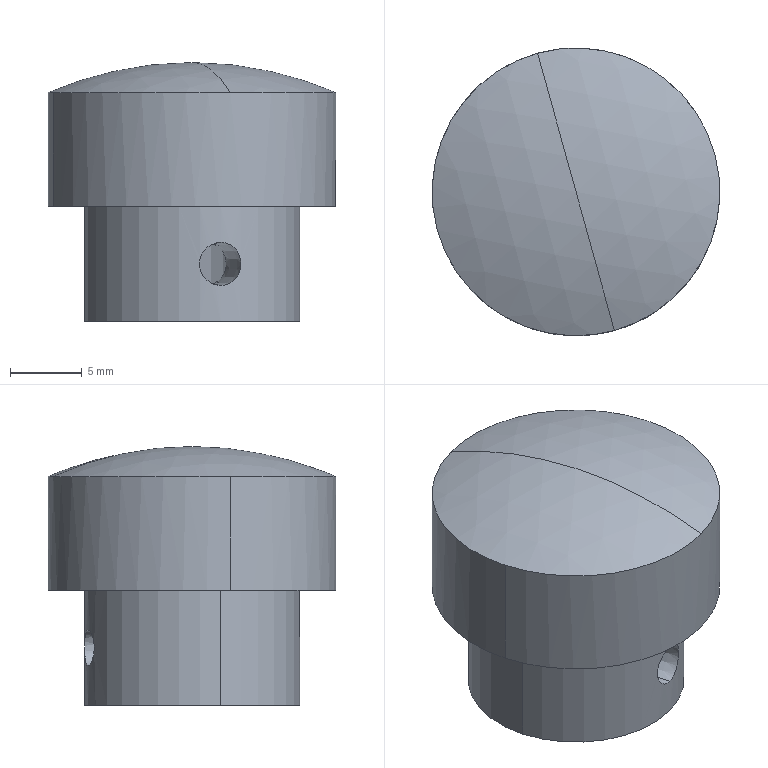Component | SolidWorks | 17Handle-1 | 1 solid | 16 faces | box 20 x 20 x 18 mm | volume 3748 mm3 | cone 6 | cylinder 6 | sphere 2 | plane 2 | commonest cylinder face diameters 8 x2 15 x2 20 x2
build123d program:
from build123d import *

# Parameters (mm, degrees)
SIZE_MM_DOWEL_PIN_HOLE1_D     = 8
SIZE_MM_DOWEL_PIN_HOLE1_DEPTH = 8
SIZE_MM_DOWEL_PIN_HOLE1_TIP   = 2.403


with BuildPart() as part:
    # Sketch6 → Revolve1 (revolve)
    with BuildSketch(Plane(origin=(0, 0, 0), x_dir=(0, 0, -1), z_dir=(1, 0, 0)), mode=Mode.PRIVATE) as revolve1_sk:
        with BuildLine():
            Line((-2.087, 10), (-10, 10))
            Line((-10, 10), (-10, 7.5))
            Line((-10, 7.5), (-18, 7.5))
            Line((-18, 7.5), (-18, 0))
            Line((-18, 0), (0, 0))
            ThreePointArc((0, 0), (-0.5273, 5.108), (-2.087, 10))
        make_face()
    revolve(revolve1_sk.sketch.rotate(Axis((0, 0, 0), (0, 0, 1)), 90), axis=Axis((0, 0, 0), (0, 0, 1)))

    # Size mm Dowel Pin Hole1
    with Locations(Plane.XY.offset(18)):
        with Locations((0, 0)):
            Hole(SIZE_MM_DOWEL_PIN_HOLE1_D / 2, depth=SIZE_MM_DOWEL_PIN_HOLE1_DEPTH)
            with Locations((0, 0, -(SIZE_MM_DOWEL_PIN_HOLE1_DEPTH + SIZE_MM_DOWEL_PIN_HOLE1_TIP / 2))):  # 118° drill point
                Cone(0, SIZE_MM_DOWEL_PIN_HOLE1_D / 2, SIZE_MM_DOWEL_PIN_HOLE1_TIP, mode=Mode.SUBTRACT)

    # Cut-Extrude2 cone 1 section (on through the dimple's axis) → Cut-Extrude2 (revolve, cut)
    with BuildSketch(Plane(origin=(0, 7.5, 14), x_dir=(0, 0, 1), z_dir=(1, 0, 0))):
        Polygon((0, 0), (1.5, 0), (0, 85.935), align=None)
    revolve(axis=Axis((0, 7.5, 14), (0, -1, 0)), mode=Mode.SUBTRACT)


solid = part.part

# Placed as in the assembly
solid = solid.moved(Location((33.957, 1.776, 451), (180, 0, -15.474)))
STEP:
#1=COLOUR_RGB('',0.7922,0.8196,0.9333);
#2=FILL_AREA_STYLE_COLOUR('',#1);
#3=FILL_AREA_STYLE('',(#2));
#4=SURFACE_STYLE_FILL_AREA(#3);
#5=SURFACE_SIDE_STYLE('',(#4));
#6=SURFACE_STYLE_USAGE(.BOTH.,#5);
#7=PRESENTATION_STYLE_ASSIGNMENT((#6));
#8=CARTESIAN_POINT('',(1.258,0.3545,17.156));
#9=VERTEX_POINT('',#8);
#10=CARTESIAN_POINT('',(1.258,0.3545,17.253));
#11=VERTEX_POINT('',#10);
#12=CARTESIAN_POINT('',(1.258,0.3545,17.156));
#13=CARTESIAN_POINT('',(1.252,0.3528,17.156));
#14=CARTESIAN_POINT('',(1.246,0.3509,17.157));
#15=CARTESIAN_POINT('',(1.235,0.347,17.162));
#16=CARTESIAN_POINT('',(1.23,0.3451,17.166));
#17=CARTESIAN_POINT('',(1.223,0.3425,17.173));
#18=CARTESIAN_POINT('',(1.221,0.3417,17.175));
#19=CARTESIAN_POINT('',(1.218,0.3403,17.18));
#20=CARTESIAN_POINT('',(1.217,0.3396,17.183));
#21=CARTESIAN_POINT('',(1.213,0.3381,17.192));
#22=CARTESIAN_POINT('',(1.212,0.3376,17.198));
#23=CARTESIAN_POINT('',(1.212,0.3375,17.211));
#24=CARTESIAN_POINT('',(1.213,0.3381,17.217));
#25=CARTESIAN_POINT('',(1.218,0.3401,17.229));
#26=CARTESIAN_POINT('',(1.221,0.3416,17.235));
#27=CARTESIAN_POINT('',(1.228,0.3442,17.241));
#28=CARTESIAN_POINT('',(1.23,0.3451,17.243));
#29=CARTESIAN_POINT('',(1.235,0.347,17.247));
#30=CARTESIAN_POINT('',(1.237,0.348,17.249));
#31=CARTESIAN_POINT('',(1.246,0.3509,17.252));
#32=CARTESIAN_POINT('',(1.252,0.3528,17.253));
#33=CARTESIAN_POINT('',(1.258,0.3545,17.253));
#34=B_SPLINE_CURVE_WITH_KNOTS('',3,(#12,#13,#14,#15,#16,#17,#18,#19,#20,#21,#22,#23,#24,#25,#26,#27,#28,#29,#30,#31,#32,#33),.UNSPECIFIED.,.F.,.F.,(4,2,2,2,2,2,2,2,2,2,4),(0.004899,0.005384,0.005868,0.006111,0.006353,0.006838,0.007323,0.007808,0.00805,0.008293,0.008778),.UNSPECIFIED.);
#35=EDGE_CURVE('',#9,#11,#34,.T.);
#36=ORIENTED_EDGE('',*,*,#35,.T.);
#37=CARTESIAN_POINT('',(1.295,0.2217,17.256));
#38=VERTEX_POINT('',#37);
#39=CARTESIAN_POINT('',(1.416,-0.2146,17.264));
#40=DIRECTION('',(0.2668,-0.9636,0.01745));
#41=VECTOR('',#40,39.37);
#42=LINE('',#39,#41);
#43=EDGE_CURVE('',#11,#38,#42,.T.);
#44=ORIENTED_EDGE('',*,*,#43,.T.);
#45=CARTESIAN_POINT('',(1.295,0.2217,17.154));
#46=VERTEX_POINT('',#45);
#47=CARTESIAN_POINT('',(1.295,0.2217,17.154));
#48=CARTESIAN_POINT('',(1.292,0.2208,17.154));
#49=CARTESIAN_POINT('',(1.288,0.2198,17.154));
#50=CARTESIAN_POINT('',(1.282,0.2176,17.155));
#51=CARTESIAN_POINT('',(1.279,0.2164,17.156));
#52=CARTESIAN_POINT('',(1.27,0.2128,17.16));
#53=CARTESIAN_POINT('',(1.265,0.2103,17.164));
#54=CARTESIAN_POINT('',(1.257,0.2056,17.173));
#55=CARTESIAN_POINT('',(1.253,0.2035,17.179));
#56=CARTESIAN_POINT('',(1.249,0.2006,17.191));
#57=CARTESIAN_POINT('',(1.248,0.1997,17.198));
#58=CARTESIAN_POINT('',(1.248,0.1997,17.208));
#59=CARTESIAN_POINT('',(1.248,0.1999,17.211));
#60=CARTESIAN_POINT('',(1.249,0.2007,17.218));
#61=CARTESIAN_POINT('',(1.25,0.2013,17.221));
#62=CARTESIAN_POINT('',(1.253,0.2035,17.231));
#63=CARTESIAN_POINT('',(1.257,0.2056,17.236));
#64=CARTESIAN_POINT('',(1.263,0.2091,17.243));
#65=CARTESIAN_POINT('',(1.266,0.2103,17.245));
#66=CARTESIAN_POINT('',(1.271,0.2128,17.249));
#67=CARTESIAN_POINT('',(1.273,0.2141,17.251));
#68=CARTESIAN_POINT('',(1.282,0.2177,17.255));
#69=CARTESIAN_POINT('',(1.288,0.2199,17.256));
#70=CARTESIAN_POINT('',(1.295,0.2217,17.256));
#71=B_SPLINE_CURVE_WITH_KNOTS('',3,(#47,#48,#49,#50,#51,#52,#53,#54,#55,#56,#57,#58,#59,#60,#61,#62,#63,#64,#65,#66,#67,#68,#69,#70),.UNSPECIFIED.,.F.,.F.,(4,2,2,2,2,2,2,2,2,2,2,4),(0.005208,0.005464,0.00572,0.006232,0.006744,0.007256,0.007512,0.007768,0.00828,0.008536,0.008792,0.009304),.UNSPECIFIED.);
#72=EDGE_CURVE('',#46,#38,#71,.T.);
#73=ORIENTED_EDGE('',*,*,#72,.F.);
#74=CARTESIAN_POINT('',(1.416,-0.2146,17.146));
#75=DIRECTION('',(0.2668,-0.9636,-0.01745));
#76=VECTOR('',#75,39.37);
#77=LINE('',#74,#76);
#78=EDGE_CURVE('',#9,#46,#77,.T.);
#79=ORIENTED_EDGE('',*,*,#78,.F.);
#80=EDGE_LOOP('',(#36,#44,#73,#79));
#81=FACE_OUTER_BOUND('',#80,.T.);
#82=CARTESIAN_POINT('',(1.416,-0.2146,17.205));
#83=DIRECTION('',(0.2668,-0.9637,0.));
#84=DIRECTION('',(0.,0.,-1.));
#85=AXIS2_PLACEMENT_3D('',#82,#83,#84);
#86=CONICAL_SURFACE('',#85,0.05906,0.01745);
#87=ADVANCED_FACE('',(#81),#86,.F.);
#88=CARTESIAN_POINT('',(1.379,-0.08185,17.261));
#89=VERTEX_POINT('',#88);
#90=CARTESIAN_POINT('',(1.379,-0.08185,17.148));
#91=VERTEX_POINT('',#90);
#92=CARTESIAN_POINT('',(1.379,-0.08185,17.261));
#93=CARTESIAN_POINT('',(1.372,-0.08383,17.261));
#94=CARTESIAN_POINT('',(1.364,-0.08529,17.26));
#95=CARTESIAN_POINT('',(1.354,-0.08665,17.256));
#96=CARTESIAN_POINT('',(1.351,-0.08697,17.254));
#97=CARTESIAN_POINT('',(1.345,-0.0874,17.25));
#98=CARTESIAN_POINT('',(1.342,-0.08751,17.247));
#99=CARTESIAN_POINT('',(1.334,-0.08762,17.24));
#100=CARTESIAN_POINT('',(1.329,-0.0874,17.233));
#101=CARTESIAN_POINT('',(1.325,-0.0871,17.223));
#102=CARTESIAN_POINT('',(1.324,-0.087,17.219));
#103=CARTESIAN_POINT('',(1.322,-0.08686,17.212));
#104=CARTESIAN_POINT('',(1.322,-0.08682,17.208));
#105=CARTESIAN_POINT('',(1.322,-0.08682,17.201));
#106=CARTESIAN_POINT('',(1.322,-0.08686,17.197));
#107=CARTESIAN_POINT('',(1.324,-0.087,17.19));
#108=CARTESIAN_POINT('',(1.325,-0.0871,17.186));
#109=CARTESIAN_POINT('',(1.329,-0.0874,17.176));
#110=CARTESIAN_POINT('',(1.334,-0.08762,17.17));
#111=CARTESIAN_POINT('',(1.342,-0.08751,17.162));
#112=CARTESIAN_POINT('',(1.345,-0.0874,17.16));
#113=CARTESIAN_POINT('',(1.351,-0.08697,17.156));
#114=CARTESIAN_POINT('',(1.354,-0.08665,17.154));
#115=CARTESIAN_POINT('',(1.361,-0.08575,17.151));
#116=CARTESIAN_POINT('',(1.365,-0.08515,17.15));
#117=CARTESIAN_POINT('',(1.372,-0.08371,17.148));
#118=CARTESIAN_POINT('',(1.375,-0.08285,17.148));
#119=CARTESIAN_POINT('',(1.379,-0.08185,17.148));
#120=B_SPLINE_CURVE_WITH_KNOTS('',3,(#92,#93,#94,#95,#96,#97,#98,#99,#100,#101,#102,#103,#104,#105,#106,#107,#108,#109,#110,#111,#112,#113,#114,#115,#116,#117,#118,#119),.UNSPECIFIED.,.F.,.F.,(4,2,2,2,2,2,2,2,2,2,2,2,2,4),(0.007846,0.008413,0.008696,0.008979,0.009545,0.009829,0.01011,0.01039,0.01068,0.01124,0.01153,0.01181,0.01209,0.01238),.UNSPECIFIED.);
#121=EDGE_CURVE('',#89,#91,#120,.T.);
#122=ORIENTED_EDGE('',*,*,#121,.F.);
#123=CARTESIAN_POINT('',(1.416,-0.2146,17.264));
#124=VERTEX_POINT('',#123);
#125=CARTESIAN_POINT('',(1.416,-0.2146,17.264));
#126=DIRECTION('',(0.2668,-0.9636,0.01745));
#127=VECTOR('',#126,39.37);
#128=LINE('',#125,#127);
#129=EDGE_CURVE('',#89,#124,#128,.T.);
#130=ORIENTED_EDGE('',*,*,#129,.T.);
#131=CARTESIAN_POINT('',(1.416,-0.2146,17.146));
#132=VERTEX_POINT('',#131);
#133=CARTESIAN_POINT('',(1.416,-0.2146,17.264));
#134=CARTESIAN_POINT('',(1.408,-0.2167,17.264));
#135=CARTESIAN_POINT('',(1.401,-0.2185,17.262));
#136=CARTESIAN_POINT('',(1.387,-0.2212,17.256));
#137=CARTESIAN_POINT('',(1.38,-0.2222,17.252));
#138=CARTESIAN_POINT('',(1.369,-0.2236,17.241));
#139=CARTESIAN_POINT('',(1.365,-0.224,17.234));
#140=CARTESIAN_POINT('',(1.36,-0.2244,17.224));
#141=CARTESIAN_POINT('',(1.359,-0.2245,17.22));
#142=CARTESIAN_POINT('',(1.358,-0.2246,17.212));
#143=CARTESIAN_POINT('',(1.357,-0.2246,17.209));
#144=CARTESIAN_POINT('',(1.357,-0.2246,17.201));
#145=CARTESIAN_POINT('',(1.358,-0.2246,17.197));
#146=CARTESIAN_POINT('',(1.359,-0.2245,17.189));
#147=CARTESIAN_POINT('',(1.36,-0.2244,17.186));
#148=CARTESIAN_POINT('',(1.365,-0.224,17.175));
#149=CARTESIAN_POINT('',(1.369,-0.2236,17.168));
#150=CARTESIAN_POINT('',(1.377,-0.2226,17.16));
#151=CARTESIAN_POINT('',(1.38,-0.2221,17.158));
#152=CARTESIAN_POINT('',(1.387,-0.2211,17.153));
#153=CARTESIAN_POINT('',(1.39,-0.2205,17.152));
#154=CARTESIAN_POINT('',(1.397,-0.2192,17.149));
#155=CARTESIAN_POINT('',(1.401,-0.2184,17.148));
#156=CARTESIAN_POINT('',(1.408,-0.2166,17.146));
#157=CARTESIAN_POINT('',(1.412,-0.2157,17.146));
#158=CARTESIAN_POINT('',(1.416,-0.2146,17.146));
#159=B_SPLINE_CURVE_WITH_KNOTS('',3,(#133,#134,#135,#136,#137,#138,#139,#140,#141,#142,#143,#144,#145,#146,#147,#148,#149,#150,#151,#152,#153,#154,#155,#156,#157,#158),.UNSPECIFIED.,.F.,.F.,(4,2,2,2,2,2,2,2,2,2,2,2,4),(0.008177,0.008764,0.009351,0.009938,0.01023,0.01053,0.01082,0.01111,0.0117,0.01199,0.01229,0.01258,0.01287),.UNSPECIFIED.);
#160=EDGE_CURVE('',#124,#132,#159,.T.);
#161=ORIENTED_EDGE('',*,*,#160,.T.);
#162=CARTESIAN_POINT('',(1.416,-0.2146,17.146));
#163=DIRECTION('',(0.2668,-0.9636,-0.01745));
#164=VECTOR('',#163,39.37);
#165=LINE('',#162,#164);
#166=EDGE_CURVE('',#91,#132,#165,.T.);
#167=ORIENTED_EDGE('',*,*,#166,.F.);
#168=EDGE_LOOP('',(#122,#130,#161,#167));
#169=FACE_OUTER_BOUND('',#168,.T.);
#170=CARTESIAN_POINT('',(1.416,-0.2146,17.205));
#171=DIRECTION('',(0.2668,-0.9637,0.));
#172=DIRECTION('',(0.,0.,-1.));
#173=AXIS2_PLACEMENT_3D('',#170,#171,#172);
#174=CONICAL_SURFACE('',#173,0.05906,0.01745);
#175=ADVANCED_FACE('',(#169),#174,.F.);
#176=ORIENTED_EDGE('',*,*,#72,.T.);
#177=CARTESIAN_POINT('',(1.295,0.2217,17.256));
#178=CARTESIAN_POINT('',(1.301,0.2235,17.256));
#179=CARTESIAN_POINT('',(1.308,0.2249,17.255));
#180=CARTESIAN_POINT('',(1.317,0.2262,17.251));
#181=CARTESIAN_POINT('',(1.32,0.2265,17.249));
#182=CARTESIAN_POINT('',(1.326,0.227,17.245));
#183=CARTESIAN_POINT('',(1.329,0.2272,17.243));
#184=CARTESIAN_POINT('',(1.336,0.2275,17.236));
#185=CARTESIAN_POINT('',(1.34,0.2274,17.231));
#186=CARTESIAN_POINT('',(1.344,0.2273,17.221));
#187=CARTESIAN_POINT('',(1.345,0.2272,17.218));
#188=CARTESIAN_POINT('',(1.346,0.2271,17.212));
#189=CARTESIAN_POINT('',(1.347,0.2271,17.208));
#190=CARTESIAN_POINT('',(1.347,0.2271,17.198));
#191=CARTESIAN_POINT('',(1.345,0.2272,17.191));
#192=CARTESIAN_POINT('',(1.34,0.2274,17.179));
#193=CARTESIAN_POINT('',(1.336,0.2275,17.173));
#194=CARTESIAN_POINT('',(1.329,0.2272,17.166));
#195=CARTESIAN_POINT('',(1.326,0.227,17.164));
#196=CARTESIAN_POINT('',(1.32,0.2265,17.16));
#197=CARTESIAN_POINT('',(1.317,0.2262,17.159));
#198=CARTESIAN_POINT('',(1.308,0.2249,17.155));
#199=CARTESIAN_POINT('',(1.301,0.2235,17.154));
#200=CARTESIAN_POINT('',(1.295,0.2217,17.154));
#201=B_SPLINE_CURVE_WITH_KNOTS('',3,(#177,#178,#179,#180,#181,#182,#183,#184,#185,#186,#187,#188,#189,#190,#191,#192,#193,#194,#195,#196,#197,#198,#199,#200),.UNSPECIFIED.,.F.,.F.,(4,2,2,2,2,2,2,2,2,2,2,4),(0.001112,0.001624,0.00188,0.002136,0.002648,0.002904,0.00316,0.003672,0.004184,0.00444,0.004696,0.005208),.UNSPECIFIED.);
#202=EDGE_CURVE('',#38,#46,#201,.T.);
#203=ORIENTED_EDGE('',*,*,#202,.T.);
#204=EDGE_LOOP('',(#176,#203));
#205=FACE_BOUND('',#204,.T.);
#206=CARTESIAN_POINT('',(1.185,0.0279,17.362));
#207=VERTEX_POINT('',#206);
#208=CARTESIAN_POINT('',(1.489,0.1119,17.362));
#209=VERTEX_POINT('',#208);
#210=CARTESIAN_POINT('',(1.337,0.06992,17.362));
#211=DIRECTION('',(0.,0.,-1.));
#212=DIRECTION('',(0.9637,0.2668,0.));
#213=AXIS2_PLACEMENT_3D('',#210,#211,#212);
#214=CIRCLE('',#213,0.1575);
#215=EDGE_CURVE('',#207,#209,#214,.T.);
#216=ORIENTED_EDGE('',*,*,#215,.F.);
#217=CARTESIAN_POINT('',(1.185,0.0279,17.047));
#218=VERTEX_POINT('',#217);
#219=CARTESIAN_POINT('',(1.185,0.0279,17.047));
#220=DIRECTION('',(0.,0.,-1.));
#221=VECTOR('',#220,39.37);
#222=LINE('',#219,#221);
#223=EDGE_CURVE('',#207,#218,#222,.T.);
#224=ORIENTED_EDGE('',*,*,#223,.T.);
#225=CARTESIAN_POINT('',(1.489,0.1119,17.047));
#226=VERTEX_POINT('',#225);
#227=CARTESIAN_POINT('',(1.337,0.06992,17.047));
#228=DIRECTION('',(0.,0.,-1.));
#229=DIRECTION('',(0.9637,0.2668,0.));
#230=AXIS2_PLACEMENT_3D('',#227,#228,#229);
#231=CIRCLE('',#230,0.1575);
#232=EDGE_CURVE('',#218,#226,#231,.T.);
#233=ORIENTED_EDGE('',*,*,#232,.T.);
#234=CARTESIAN_POINT('',(1.489,0.1119,17.047));
#235=DIRECTION('',(0.,0.,-1.));
#236=VECTOR('',#235,39.37);
#237=LINE('',#234,#236);
#238=EDGE_CURVE('',#209,#226,#237,.T.);
#239=ORIENTED_EDGE('',*,*,#238,.F.);
#240=EDGE_LOOP('',(#216,#224,#233,#239));
#241=FACE_OUTER_BOUND('',#240,.T.);
#242=CARTESIAN_POINT('',(1.337,0.06992,17.047));
#243=DIRECTION('',(0.,0.,-1.));
#244=DIRECTION('',(0.9637,0.2668,0.));
#245=AXIS2_PLACEMENT_3D('',#242,#243,#244);
#246=CYLINDRICAL_SURFACE('',#245,0.1575);
#247=ADVANCED_FACE('',(#205,#241),#246,.F.);
#248=CARTESIAN_POINT('',(1.337,0.06992,17.457));
#249=VERTEX_POINT('',#248);
#250=CARTESIAN_POINT('',(1.489,0.1119,17.362));
#251=DIRECTION('',(0.8261,0.2287,-0.515));
#252=VECTOR('',#251,39.37);
#253=LINE('',#250,#252);
#254=EDGE_CURVE('',#249,#209,#253,.T.);
#255=ORIENTED_EDGE('',*,*,#254,.F.);
#256=CARTESIAN_POINT('',(1.185,0.0279,17.362));
#257=DIRECTION('',(-0.8261,-0.2287,-0.515));
#258=VECTOR('',#257,39.37);
#259=LINE('',#256,#258);
#260=EDGE_CURVE('',#249,#207,#259,.T.);
#261=ORIENTED_EDGE('',*,*,#260,.T.);
#262=ORIENTED_EDGE('',*,*,#215,.T.);
#263=EDGE_LOOP('',(#255,#261,#262));
#264=FACE_OUTER_BOUND('',#263,.T.);
#265=CARTESIAN_POINT('',(1.337,0.06992,17.362));
#266=DIRECTION('',(0.,0.,-1.));
#267=DIRECTION('',(0.9637,0.2668,0.));
#268=AXIS2_PLACEMENT_3D('',#265,#266,#267);
#269=CONICAL_SURFACE('',#268,0.1575,1.03);
#270=ADVANCED_FACE('',(#264),#269,.F.);
#271=CARTESIAN_POINT('',(1.416,-0.2146,17.146));
#272=CARTESIAN_POINT('',(1.423,-0.2126,17.146));
#273=CARTESIAN_POINT('',(1.431,-0.2102,17.147));
#274=CARTESIAN_POINT('',(1.441,-0.2066,17.152));
#275=CARTESIAN_POINT('',(1.444,-0.2053,17.154));
#276=CARTESIAN_POINT('',(1.45,-0.2029,17.158));
#277=CARTESIAN_POINT('',(1.453,-0.2018,17.16));
#278=CARTESIAN_POINT('',(1.46,-0.1985,17.168));
#279=CARTESIAN_POINT('',(1.464,-0.1965,17.175));
#280=CARTESIAN_POINT('',(1.47,-0.1939,17.189));
#281=CARTESIAN_POINT('',(1.471,-0.1932,17.197));
#282=CARTESIAN_POINT('',(1.471,-0.1932,17.209));
#283=CARTESIAN_POINT('',(1.471,-0.1934,17.212));
#284=CARTESIAN_POINT('',(1.469,-0.1941,17.22));
#285=CARTESIAN_POINT('',(1.468,-0.1946,17.224));
#286=CARTESIAN_POINT('',(1.465,-0.1959,17.231));
#287=CARTESIAN_POINT('',(1.464,-0.1967,17.234));
#288=CARTESIAN_POINT('',(1.46,-0.1985,17.241));
#289=CARTESIAN_POINT('',(1.458,-0.1996,17.244));
#290=CARTESIAN_POINT('',(1.45,-0.2029,17.252));
#291=CARTESIAN_POINT('',(1.444,-0.2053,17.256));
#292=CARTESIAN_POINT('',(1.434,-0.209,17.261));
#293=CARTESIAN_POINT('',(1.43,-0.2102,17.262));
#294=CARTESIAN_POINT('',(1.423,-0.2125,17.263));
#295=CARTESIAN_POINT('',(1.419,-0.2136,17.264));
#296=CARTESIAN_POINT('',(1.416,-0.2146,17.264));
#297=B_SPLINE_CURVE_WITH_KNOTS('',3,(#271,#272,#273,#274,#275,#276,#277,#278,#279,#280,#281,#282,#283,#284,#285,#286,#287,#288,#289,#290,#291,#292,#293,#294,#295,#296),.UNSPECIFIED.,.F.,.F.,(4,2,2,2,2,2,2,2,2,2,2,2,4),(0.003479,0.004067,0.00436,0.004654,0.005241,0.005828,0.006122,0.006415,0.006709,0.007002,0.007589,0.007883,0.008177),.UNSPECIFIED.);
#298=EDGE_CURVE('',#132,#124,#297,.T.);
#299=ORIENTED_EDGE('',*,*,#298,.F.);
#300=ORIENTED_EDGE('',*,*,#160,.F.);
#301=EDGE_LOOP('',(#299,#300));
#302=FACE_BOUND('',#301,.T.);
#303=CARTESIAN_POINT('',(1.052,-0.008864,17.047));
#304=VERTEX_POINT('',#303);
#305=CARTESIAN_POINT('',(1.621,0.1487,17.047));
#306=VERTEX_POINT('',#305);
#307=CARTESIAN_POINT('',(1.337,0.06992,17.047));
#308=DIRECTION('',(-0.,-0.,1.));
#309=DIRECTION('',(-0.9637,-0.2668,0.));
#310=AXIS2_PLACEMENT_3D('',#307,#308,#309);
#311=CIRCLE('',#310,0.2953);
#312=EDGE_CURVE('',#304,#306,#311,.T.);
#313=ORIENTED_EDGE('',*,*,#312,.T.);
#314=CARTESIAN_POINT('',(1.621,0.1487,17.362));
#315=VERTEX_POINT('',#314);
#316=CARTESIAN_POINT('',(1.621,0.1487,17.756));
#317=DIRECTION('',(-0.,-0.,1.));
#318=VECTOR('',#317,39.37);
#319=LINE('',#316,#318);
#320=EDGE_CURVE('',#306,#315,#319,.T.);
#321=ORIENTED_EDGE('',*,*,#320,.T.);
#322=CARTESIAN_POINT('',(1.052,-0.008864,17.362));
#323=VERTEX_POINT('',#322);
#324=CARTESIAN_POINT('',(1.337,0.06992,17.362));
#325=DIRECTION('',(-0.,-0.,1.));
#326=DIRECTION('',(-0.9637,-0.2668,0.));
#327=AXIS2_PLACEMENT_3D('',#324,#325,#326);
#328=CIRCLE('',#327,0.2953);
#329=EDGE_CURVE('',#323,#315,#328,.T.);
#330=ORIENTED_EDGE('',*,*,#329,.F.);
#331=CARTESIAN_POINT('',(1.052,-0.008864,17.756));
#332=DIRECTION('',(-0.,-0.,1.));
#333=VECTOR('',#332,39.37);
#334=LINE('',#331,#333);
#335=EDGE_CURVE('',#304,#323,#334,.T.);
#336=ORIENTED_EDGE('',*,*,#335,.F.);
#337=EDGE_LOOP('',(#313,#321,#330,#336));
#338=FACE_OUTER_BOUND('',#337,.T.);
#339=CARTESIAN_POINT('',(1.337,0.06992,17.756));
#340=DIRECTION('',(-0.,-0.,1.));
#341=DIRECTION('',(-0.9637,-0.2668,0.));
#342=AXIS2_PLACEMENT_3D('',#339,#340,#341);
#343=CYLINDRICAL_SURFACE('',#342,0.2953);
#344=ADVANCED_FACE('',(#302,#338),#343,.T.);
#345=CARTESIAN_POINT('',(0.9575,-0.03513,17.362));
#346=VERTEX_POINT('',#345);
#347=CARTESIAN_POINT('',(1.716,0.175,17.362));
#348=VERTEX_POINT('',#347);
#349=CARTESIAN_POINT('',(1.337,0.06992,17.362));
#350=DIRECTION('',(-0.,-0.,1.));
#351=DIRECTION('',(-0.9637,-0.2668,0.));
#352=AXIS2_PLACEMENT_3D('',#349,#350,#351);
#353=CIRCLE('',#352,0.3937);
#354=EDGE_CURVE('',#346,#348,#353,.T.);
#355=ORIENTED_EDGE('',*,*,#354,.T.);
#356=CARTESIAN_POINT('',(1.716,0.175,17.674));
#357=VERTEX_POINT('',#356);
#358=CARTESIAN_POINT('',(1.716,0.175,17.756));
#359=DIRECTION('',(-0.,-0.,1.));
#360=VECTOR('',#359,39.37);
#361=LINE('',#358,#360);
#362=EDGE_CURVE('',#348,#357,#361,.T.);
#363=ORIENTED_EDGE('',*,*,#362,.T.);
#364=CARTESIAN_POINT('',(1.442,-0.3095,17.674));
#365=VERTEX_POINT('',#364);
#366=CARTESIAN_POINT('',(1.337,0.06992,17.674));
#367=DIRECTION('',(-0.,-0.,1.));
#368=DIRECTION('',(-0.9637,-0.2668,0.));
#369=AXIS2_PLACEMENT_3D('',#366,#367,#368);
#370=CIRCLE('',#369,0.3937);
#371=EDGE_CURVE('',#365,#357,#370,.T.);
#372=ORIENTED_EDGE('',*,*,#371,.F.);
#373=CARTESIAN_POINT('',(0.9575,-0.03513,17.674));
#374=VERTEX_POINT('',#373);
#375=CARTESIAN_POINT('',(1.337,0.06992,17.674));
#376=DIRECTION('',(-0.,-0.,1.));
#377=DIRECTION('',(-0.9637,-0.2668,0.));
#378=AXIS2_PLACEMENT_3D('',#375,#376,#377);
#379=CIRCLE('',#378,0.3937);
#380=EDGE_CURVE('',#374,#365,#379,.T.);
#381=ORIENTED_EDGE('',*,*,#380,.F.);
#382=CARTESIAN_POINT('',(0.9575,-0.03513,17.756));
#383=DIRECTION('',(-0.,-0.,1.));
#384=VECTOR('',#383,39.37);
#385=LINE('',#382,#384);
#386=EDGE_CURVE('',#346,#374,#385,.T.);
#387=ORIENTED_EDGE('',*,*,#386,.F.);
#388=EDGE_LOOP('',(#355,#363,#372,#381,#387));
#389=FACE_OUTER_BOUND('',#388,.T.);
#390=CARTESIAN_POINT('',(1.337,0.06992,17.756));
#391=DIRECTION('',(-0.,-0.,1.));
#392=DIRECTION('',(-0.9637,-0.2668,0.));
#393=AXIS2_PLACEMENT_3D('',#390,#391,#392);
#394=CYLINDRICAL_SURFACE('',#393,0.3937);
#395=ADVANCED_FACE('',(#389),#394,.T.);
#396=CARTESIAN_POINT('',(1.232,0.4493,17.674));
#397=VERTEX_POINT('',#396);
#398=CARTESIAN_POINT('',(1.337,0.06992,17.674));
#399=DIRECTION('',(-0.,-0.,1.));
#400=DIRECTION('',(-0.9637,-0.2668,0.));
#401=AXIS2_PLACEMENT_3D('',#398,#399,#400);
#402=CIRCLE('',#401,0.3937);
#403=EDGE_CURVE('',#397,#374,#402,.T.);
#404=ORIENTED_EDGE('',*,*,#403,.T.);
#405=ORIENTED_EDGE('',*,*,#380,.T.);
#406=CARTESIAN_POINT('',(1.337,0.06992,17.756));
#407=VERTEX_POINT('',#406);
#408=CARTESIAN_POINT('',(1.337,0.06992,16.772));
#409=DIRECTION('',(-0.9637,-0.2668,-0.));
#410=DIRECTION('',(0.2668,-0.9637,0.));
#411=AXIS2_PLACEMENT_3D('',#408,#409,#410);
#412=CIRCLE('',#411,0.9843);
#413=EDGE_CURVE('',#365,#407,#412,.T.);
#414=ORIENTED_EDGE('',*,*,#413,.T.);
#415=CARTESIAN_POINT('',(1.337,0.06992,16.772));
#416=DIRECTION('',(0.9637,0.2668,0.));
#417=DIRECTION('',(-0.2668,0.9637,0.));
#418=AXIS2_PLACEMENT_3D('',#415,#416,#417);
#419=CIRCLE('',#418,0.9843);
#420=EDGE_CURVE('',#397,#407,#419,.T.);
#421=ORIENTED_EDGE('',*,*,#420,.F.);
#422=EDGE_LOOP('',(#404,#405,#414,#421));
#423=FACE_OUTER_BOUND('',#422,.T.);
#424=CARTESIAN_POINT('',(1.337,0.06992,16.772));
#425=DIRECTION('',(-0.9637,-0.2668,-0.));
#426=DIRECTION('',(-0.2668,0.9637,0.));
#427=AXIS2_PLACEMENT_3D('',#424,#425,#426);
#428=SPHERICAL_SURFACE('',#427,0.9843);
#429=ADVANCED_FACE('',(#423),#428,.T.);
#430=ORIENTED_EDGE('',*,*,#413,.F.);
#431=ORIENTED_EDGE('',*,*,#371,.T.);
#432=CARTESIAN_POINT('',(1.337,0.06992,17.674));
#433=DIRECTION('',(-0.,-0.,1.));
#434=DIRECTION('',(-0.9637,-0.2668,0.));
#435=AXIS2_PLACEMENT_3D('',#432,#433,#434);
#436=CIRCLE('',#435,0.3937);
#437=EDGE_CURVE('',#357,#397,#436,.T.);
#438=ORIENTED_EDGE('',*,*,#437,.T.);
#439=ORIENTED_EDGE('',*,*,#420,.T.);
#440=EDGE_LOOP('',(#430,#431,#438,#439));
#441=FACE_OUTER_BOUND('',#440,.T.);
#442=CARTESIAN_POINT('',(1.337,0.06992,16.772));
#443=DIRECTION('',(-0.9637,-0.2668,-0.));
#444=DIRECTION('',(-0.2668,0.9637,0.));
#445=AXIS2_PLACEMENT_3D('',#442,#443,#444);
#446=SPHERICAL_SURFACE('',#445,0.9843);
#447=ADVANCED_FACE('',(#441),#446,.T.);
#448=ORIENTED_EDGE('',*,*,#362,.F.);
#449=CARTESIAN_POINT('',(1.337,0.06992,17.362));
#450=DIRECTION('',(-0.,-0.,1.));
#451=DIRECTION('',(-0.9637,-0.2668,0.));
#452=AXIS2_PLACEMENT_3D('',#449,#450,#451);
#453=CIRCLE('',#452,0.3937);
#454=EDGE_CURVE('',#348,#346,#453,.T.);
#455=ORIENTED_EDGE('',*,*,#454,.T.);
#456=ORIENTED_EDGE('',*,*,#386,.T.);
#457=ORIENTED_EDGE('',*,*,#403,.F.);
#458=ORIENTED_EDGE('',*,*,#437,.F.);
#459=EDGE_LOOP('',(#448,#455,#456,#457,#458));
#460=FACE_OUTER_BOUND('',#459,.T.);
#461=CARTESIAN_POINT('',(1.337,0.06992,17.756));
#462=DIRECTION('',(-0.,-0.,1.));
#463=DIRECTION('',(-0.9637,-0.2668,0.));
#464=AXIS2_PLACEMENT_3D('',#461,#462,#463);
#465=CYLINDRICAL_SURFACE('',#464,0.3937);
#466=ADVANCED_FACE('',(#460),#465,.T.);
#467=ORIENTED_EDGE('',*,*,#329,.T.);
#468=CARTESIAN_POINT('',(1.337,0.06992,17.362));
#469=DIRECTION('',(-0.,-0.,1.));
#470=DIRECTION('',(-0.9637,-0.2668,0.));
#471=AXIS2_PLACEMENT_3D('',#468,#469,#470);
#472=CIRCLE('',#471,0.2953);
#473=EDGE_CURVE('',#315,#323,#472,.T.);
#474=ORIENTED_EDGE('',*,*,#473,.T.);
#475=EDGE_LOOP('',(#467,#474));
#476=FACE_BOUND('',#475,.T.);
#477=ORIENTED_EDGE('',*,*,#354,.F.);
#478=ORIENTED_EDGE('',*,*,#454,.F.);
#479=EDGE_LOOP('',(#477,#478));
#480=FACE_OUTER_BOUND('',#479,.T.);
#481=CARTESIAN_POINT('',(1.442,-0.3095,17.362));
#482=DIRECTION('',(0.,0.,-1.));
#483=DIRECTION('',(0.9637,0.2668,0.));
#484=AXIS2_PLACEMENT_3D('',#481,#482,#483);
#485=PLANE('',#484);
#486=ADVANCED_FACE('',(#476,#480),#485,.T.);
#487=ORIENTED_EDGE('',*,*,#320,.F.);
#488=CARTESIAN_POINT('',(1.337,0.06992,17.047));
#489=DIRECTION('',(-0.,-0.,1.));
#490=DIRECTION('',(-0.9637,-0.2668,0.));
#491=AXIS2_PLACEMENT_3D('',#488,#489,#490);
#492=CIRCLE('',#491,0.2953);
#493=EDGE_CURVE('',#306,#304,#492,.T.);
#494=ORIENTED_EDGE('',*,*,#493,.T.);
#495=ORIENTED_EDGE('',*,*,#335,.T.);
#496=ORIENTED_EDGE('',*,*,#473,.F.);
#497=EDGE_LOOP('',(#487,#494,#495,#496));
#498=FACE_OUTER_BOUND('',#497,.T.);
#499=ORIENTED_EDGE('',*,*,#35,.F.);
#500=CARTESIAN_POINT('',(1.258,0.3545,17.253));
#501=CARTESIAN_POINT('',(1.264,0.3562,17.253));
#502=CARTESIAN_POINT('',(1.271,0.3577,17.252));
#503=CARTESIAN_POINT('',(1.282,0.3601,17.247));
#504=CARTESIAN_POINT('',(1.287,0.3611,17.244));
#505=CARTESIAN_POINT('',(1.296,0.3624,17.235));
#506=CARTESIAN_POINT('',(1.3,0.3629,17.229));
#507=CARTESIAN_POINT('',(1.305,0.3635,17.217));
#508=CARTESIAN_POINT('',(1.306,0.3636,17.211));
#509=CARTESIAN_POINT('',(1.306,0.3636,17.201));
#510=CARTESIAN_POINT('',(1.306,0.3636,17.198));
#511=CARTESIAN_POINT('',(1.305,0.3634,17.192));
#512=CARTESIAN_POINT('',(1.304,0.3633,17.189));
#513=CARTESIAN_POINT('',(1.3,0.3629,17.18));
#514=CARTESIAN_POINT('',(1.296,0.3624,17.175));
#515=CARTESIAN_POINT('',(1.287,0.3611,17.166));
#516=CARTESIAN_POINT('',(1.282,0.3601,17.162));
#517=CARTESIAN_POINT('',(1.271,0.3577,17.157));
#518=CARTESIAN_POINT('',(1.264,0.3562,17.156));
#519=CARTESIAN_POINT('',(1.258,0.3545,17.156));
#520=B_SPLINE_CURVE_WITH_KNOTS('',3,(#500,#501,#502,#503,#504,#505,#506,#507,#508,#509,#510,#511,#512,#513,#514,#515,#516,#517,#518,#519),.UNSPECIFIED.,.F.,.F.,(4,2,2,2,2,2,2,2,2,4),(0.001017,0.001502,0.001988,0.002473,0.002958,0.003201,0.003443,0.003928,0.004413,0.004899),.UNSPECIFIED.);
#521=EDGE_CURVE('',#11,#9,#520,.T.);
#522=ORIENTED_EDGE('',*,*,#521,.F.);
#523=EDGE_LOOP('',(#499,#522));
#524=FACE_BOUND('',#523,.T.);
#525=CARTESIAN_POINT('',(1.337,0.06992,17.756));
#526=DIRECTION('',(-0.,-0.,1.));
#527=DIRECTION('',(-0.9637,-0.2668,0.));
#528=AXIS2_PLACEMENT_3D('',#525,#526,#527);
#529=CYLINDRICAL_SURFACE('',#528,0.2953);
#530=ADVANCED_FACE('',(#498,#524),#529,.T.);
#531=CARTESIAN_POINT('',(1.337,0.06992,17.047));
#532=DIRECTION('',(0.,0.,-1.));
#533=DIRECTION('',(0.9637,0.2668,0.));
#534=AXIS2_PLACEMENT_3D('',#531,#532,#533);
#535=CIRCLE('',#534,0.1575);
#536=EDGE_CURVE('',#226,#218,#535,.T.);
#537=ORIENTED_EDGE('',*,*,#536,.F.);
#538=ORIENTED_EDGE('',*,*,#232,.F.);
#539=EDGE_LOOP('',(#537,#538));
#540=FACE_BOUND('',#539,.T.);
#541=ORIENTED_EDGE('',*,*,#312,.F.);
#542=ORIENTED_EDGE('',*,*,#493,.F.);
#543=EDGE_LOOP('',(#541,#542));
#544=FACE_OUTER_BOUND('',#543,.T.);
#545=CARTESIAN_POINT('',(1.416,-0.2146,17.047));
#546=DIRECTION('',(0.,0.,-1.));
#547=DIRECTION('',(0.9637,0.2668,0.));
#548=AXIS2_PLACEMENT_3D('',#545,#546,#547);
#549=PLANE('',#548);
#550=ADVANCED_FACE('',(#540,#544),#549,.T.);
#551=ORIENTED_EDGE('',*,*,#260,.F.);
#552=ORIENTED_EDGE('',*,*,#254,.T.);
#553=CARTESIAN_POINT('',(1.337,0.06992,17.362));
#554=DIRECTION('',(0.,0.,-1.));
#555=DIRECTION('',(0.9637,0.2668,0.));
#556=AXIS2_PLACEMENT_3D('',#553,#554,#555);
#557=CIRCLE('',#556,0.1575);
#558=EDGE_CURVE('',#209,#207,#557,.T.);
#559=ORIENTED_EDGE('',*,*,#558,.T.);
#560=EDGE_LOOP('',(#551,#552,#559));
#561=FACE_OUTER_BOUND('',#560,.T.);
#562=CARTESIAN_POINT('',(1.337,0.06992,17.362));
#563=DIRECTION('',(0.,0.,-1.));
#564=DIRECTION('',(0.9637,0.2668,0.));
#565=AXIS2_PLACEMENT_3D('',#562,#563,#564);
#566=CONICAL_SURFACE('',#565,0.1575,1.03);
#567=ADVANCED_FACE('',(#561),#566,.F.);
#568=ORIENTED_EDGE('',*,*,#223,.F.);
#569=ORIENTED_EDGE('',*,*,#558,.F.);
#570=ORIENTED_EDGE('',*,*,#238,.T.);
#571=ORIENTED_EDGE('',*,*,#536,.T.);
#572=EDGE_LOOP('',(#568,#569,#570,#571));
#573=FACE_OUTER_BOUND('',#572,.T.);
#574=CARTESIAN_POINT('',(1.379,-0.08185,17.148));
#575=CARTESIAN_POINT('',(1.386,-0.07984,17.148));
#576=CARTESIAN_POINT('',(1.393,-0.07733,17.15));
#577=CARTESIAN_POINT('',(1.406,-0.07183,17.155));
#578=CARTESIAN_POINT('',(1.411,-0.06888,17.16));
#579=CARTESIAN_POINT('',(1.421,-0.06352,17.17));
#580=CARTESIAN_POINT('',(1.424,-0.06108,17.176));
#581=CARTESIAN_POINT('',(1.429,-0.05767,17.19));
#582=CARTESIAN_POINT('',(1.431,-0.05669,17.197));
#583=CARTESIAN_POINT('',(1.431,-0.05669,17.208));
#584=CARTESIAN_POINT('',(1.43,-0.05693,17.212));
#585=CARTESIAN_POINT('',(1.429,-0.05784,17.219));
#586=CARTESIAN_POINT('',(1.428,-0.05851,17.223));
#587=CARTESIAN_POINT('',(1.424,-0.0611,17.233));
#588=CARTESIAN_POINT('',(1.421,-0.06353,17.24));
#589=CARTESIAN_POINT('',(1.414,-0.06758,17.247));
#590=CARTESIAN_POINT('',(1.411,-0.06897,17.25));
#591=CARTESIAN_POINT('',(1.406,-0.0718,17.254));
#592=CARTESIAN_POINT('',(1.403,-0.07323,17.256));
#593=CARTESIAN_POINT('',(1.393,-0.07733,17.26));
#594=CARTESIAN_POINT('',(1.386,-0.07987,17.261));
#595=CARTESIAN_POINT('',(1.379,-0.08185,17.261));
#596=B_SPLINE_CURVE_WITH_KNOTS('',3,(#574,#575,#576,#577,#578,#579,#580,#581,#582,#583,#584,#585,#586,#587,#588,#589,#590,#591,#592,#593,#594,#595),.UNSPECIFIED.,.F.,.F.,(4,2,2,2,2,2,2,2,2,2,4),(0.003317,0.003883,0.004449,0.005015,0.005582,0.005865,0.006148,0.006714,0.006997,0.00728,0.007846),.UNSPECIFIED.);
#597=EDGE_CURVE('',#91,#89,#596,.T.);
#598=ORIENTED_EDGE('',*,*,#597,.T.);
#599=ORIENTED_EDGE('',*,*,#121,.T.);
#600=EDGE_LOOP('',(#598,#599));
#601=FACE_BOUND('',#600,.T.);
#602=CARTESIAN_POINT('',(1.337,0.06992,17.047));
#603=DIRECTION('',(0.,0.,-1.));
#604=DIRECTION('',(0.9637,0.2668,0.));
#605=AXIS2_PLACEMENT_3D('',#602,#603,#604);
#606=CYLINDRICAL_SURFACE('',#605,0.1575);
#607=ADVANCED_FACE('',(#573,#601),#606,.F.);
#608=ORIENTED_EDGE('',*,*,#129,.F.);
#609=ORIENTED_EDGE('',*,*,#597,.F.);
#610=ORIENTED_EDGE('',*,*,#166,.T.);
#611=ORIENTED_EDGE('',*,*,#298,.T.);
#612=EDGE_LOOP('',(#608,#609,#610,#611));
#613=FACE_OUTER_BOUND('',#612,.T.);
#614=CARTESIAN_POINT('',(1.416,-0.2146,17.205));
#615=DIRECTION('',(0.2668,-0.9637,0.));
#616=DIRECTION('',(0.,0.,-1.));
#617=AXIS2_PLACEMENT_3D('',#614,#615,#616);
#618=CONICAL_SURFACE('',#617,0.05906,0.01745);
#619=ADVANCED_FACE('',(#613),#618,.F.);
#620=ORIENTED_EDGE('',*,*,#43,.F.);
#621=ORIENTED_EDGE('',*,*,#521,.T.);
#622=ORIENTED_EDGE('',*,*,#78,.T.);
#623=ORIENTED_EDGE('',*,*,#202,.F.);
#624=EDGE_LOOP('',(#620,#621,#622,#623));
#625=FACE_OUTER_BOUND('',#624,.T.);
#626=CARTESIAN_POINT('',(1.416,-0.2146,17.205));
#627=DIRECTION('',(0.2668,-0.9637,0.));
#628=DIRECTION('',(0.,0.,-1.));
#629=AXIS2_PLACEMENT_3D('',#626,#627,#628);
#630=CONICAL_SURFACE('',#629,0.05906,0.01745);
#631=ADVANCED_FACE('',(#625),#630,.F.);
#632=CLOSED_SHELL('',(#87,#175,#247,#270,#344,#395,#429,#447,#466,#486,#530,#550,#567,#607,#619,#631));
#633=MANIFOLD_SOLID_BREP('',#632);
#634=STYLED_ITEM('',(#7),#633);
#635=(LENGTH_UNIT()NAMED_UNIT(*)SI_UNIT($,.METRE.));
#636=LENGTH_MEASURE_WITH_UNIT(LENGTH_MEASURE(0.0254),#635);
#637=DIMENSIONAL_EXPONENTS(1.,0.,0.,0.,0.,0.,0.);
#638=(CONVERSION_BASED_UNIT('',#636)LENGTH_UNIT()NAMED_UNIT(#637));
#639=UNCERTAINTY_MEASURE_WITH_UNIT(LENGTH_MEASURE(0.00001),#638,'','');
#640=(NAMED_UNIT(*)PLANE_ANGLE_UNIT()SI_UNIT($,.RADIAN.));
#641=(NAMED_UNIT(*)SI_UNIT($,.STERADIAN.)SOLID_ANGLE_UNIT());
#642=(GEOMETRIC_REPRESENTATION_CONTEXT(3)GLOBAL_UNCERTAINTY_ASSIGNED_CONTEXT((#639))GLOBAL_UNIT_ASSIGNED_CONTEXT((#638,#640,#641))REPRESENTATION_CONTEXT('',''));
#643=MECHANICAL_DESIGN_GEOMETRIC_PRESENTATION_REPRESENTATION('',(#634),#642);
#644=CARTESIAN_POINT('',(0.,0.,0.));
#645=DIRECTION('',(0.,0.,1.));
#646=DIRECTION('',(1.,0.,0.));
#647=AXIS2_PLACEMENT_3D('',#644,#645,#646);
#648=(LENGTH_UNIT()NAMED_UNIT(*)SI_UNIT($,.METRE.));
#649=LENGTH_MEASURE_WITH_UNIT(LENGTH_MEASURE(0.0254),#648);
#650=DIMENSIONAL_EXPONENTS(1.,0.,0.,0.,0.,0.,0.);
#651=(CONVERSION_BASED_UNIT('',#649)LENGTH_UNIT()NAMED_UNIT(#650));
#652=UNCERTAINTY_MEASURE_WITH_UNIT(LENGTH_MEASURE(0.00001),#651,'','');
#653=(NAMED_UNIT(*)PLANE_ANGLE_UNIT()SI_UNIT($,.RADIAN.));
#654=(NAMED_UNIT(*)SI_UNIT($,.STERADIAN.)SOLID_ANGLE_UNIT());
#655=(GEOMETRIC_REPRESENTATION_CONTEXT(3)GLOBAL_UNCERTAINTY_ASSIGNED_CONTEXT((#652))GLOBAL_UNIT_ASSIGNED_CONTEXT((#651,#653,#654))REPRESENTATION_CONTEXT('',''));
#656=ADVANCED_BREP_SHAPE_REPRESENTATION('',(#633,#647),#655);
#657=PRESENTATION_LAYER_ASSIGNMENT('','',(#634));